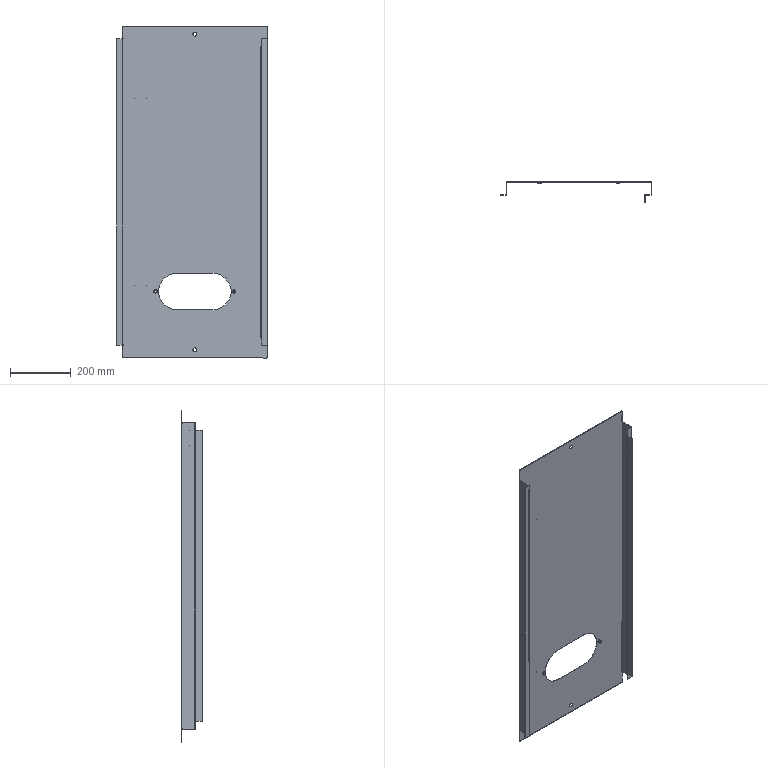Component | SolidWorks | CabinetWelding-1_TopCover-1 | 1 solid | 104 faces | volume 781534 mm3 | cylinder 52 | plane 46 | spline 6 | commonest cylinder face diameters 3 x12 1 x8 0.2 x5 2.6 x5 6 x4 11 x4 0.5 x4 13 x4